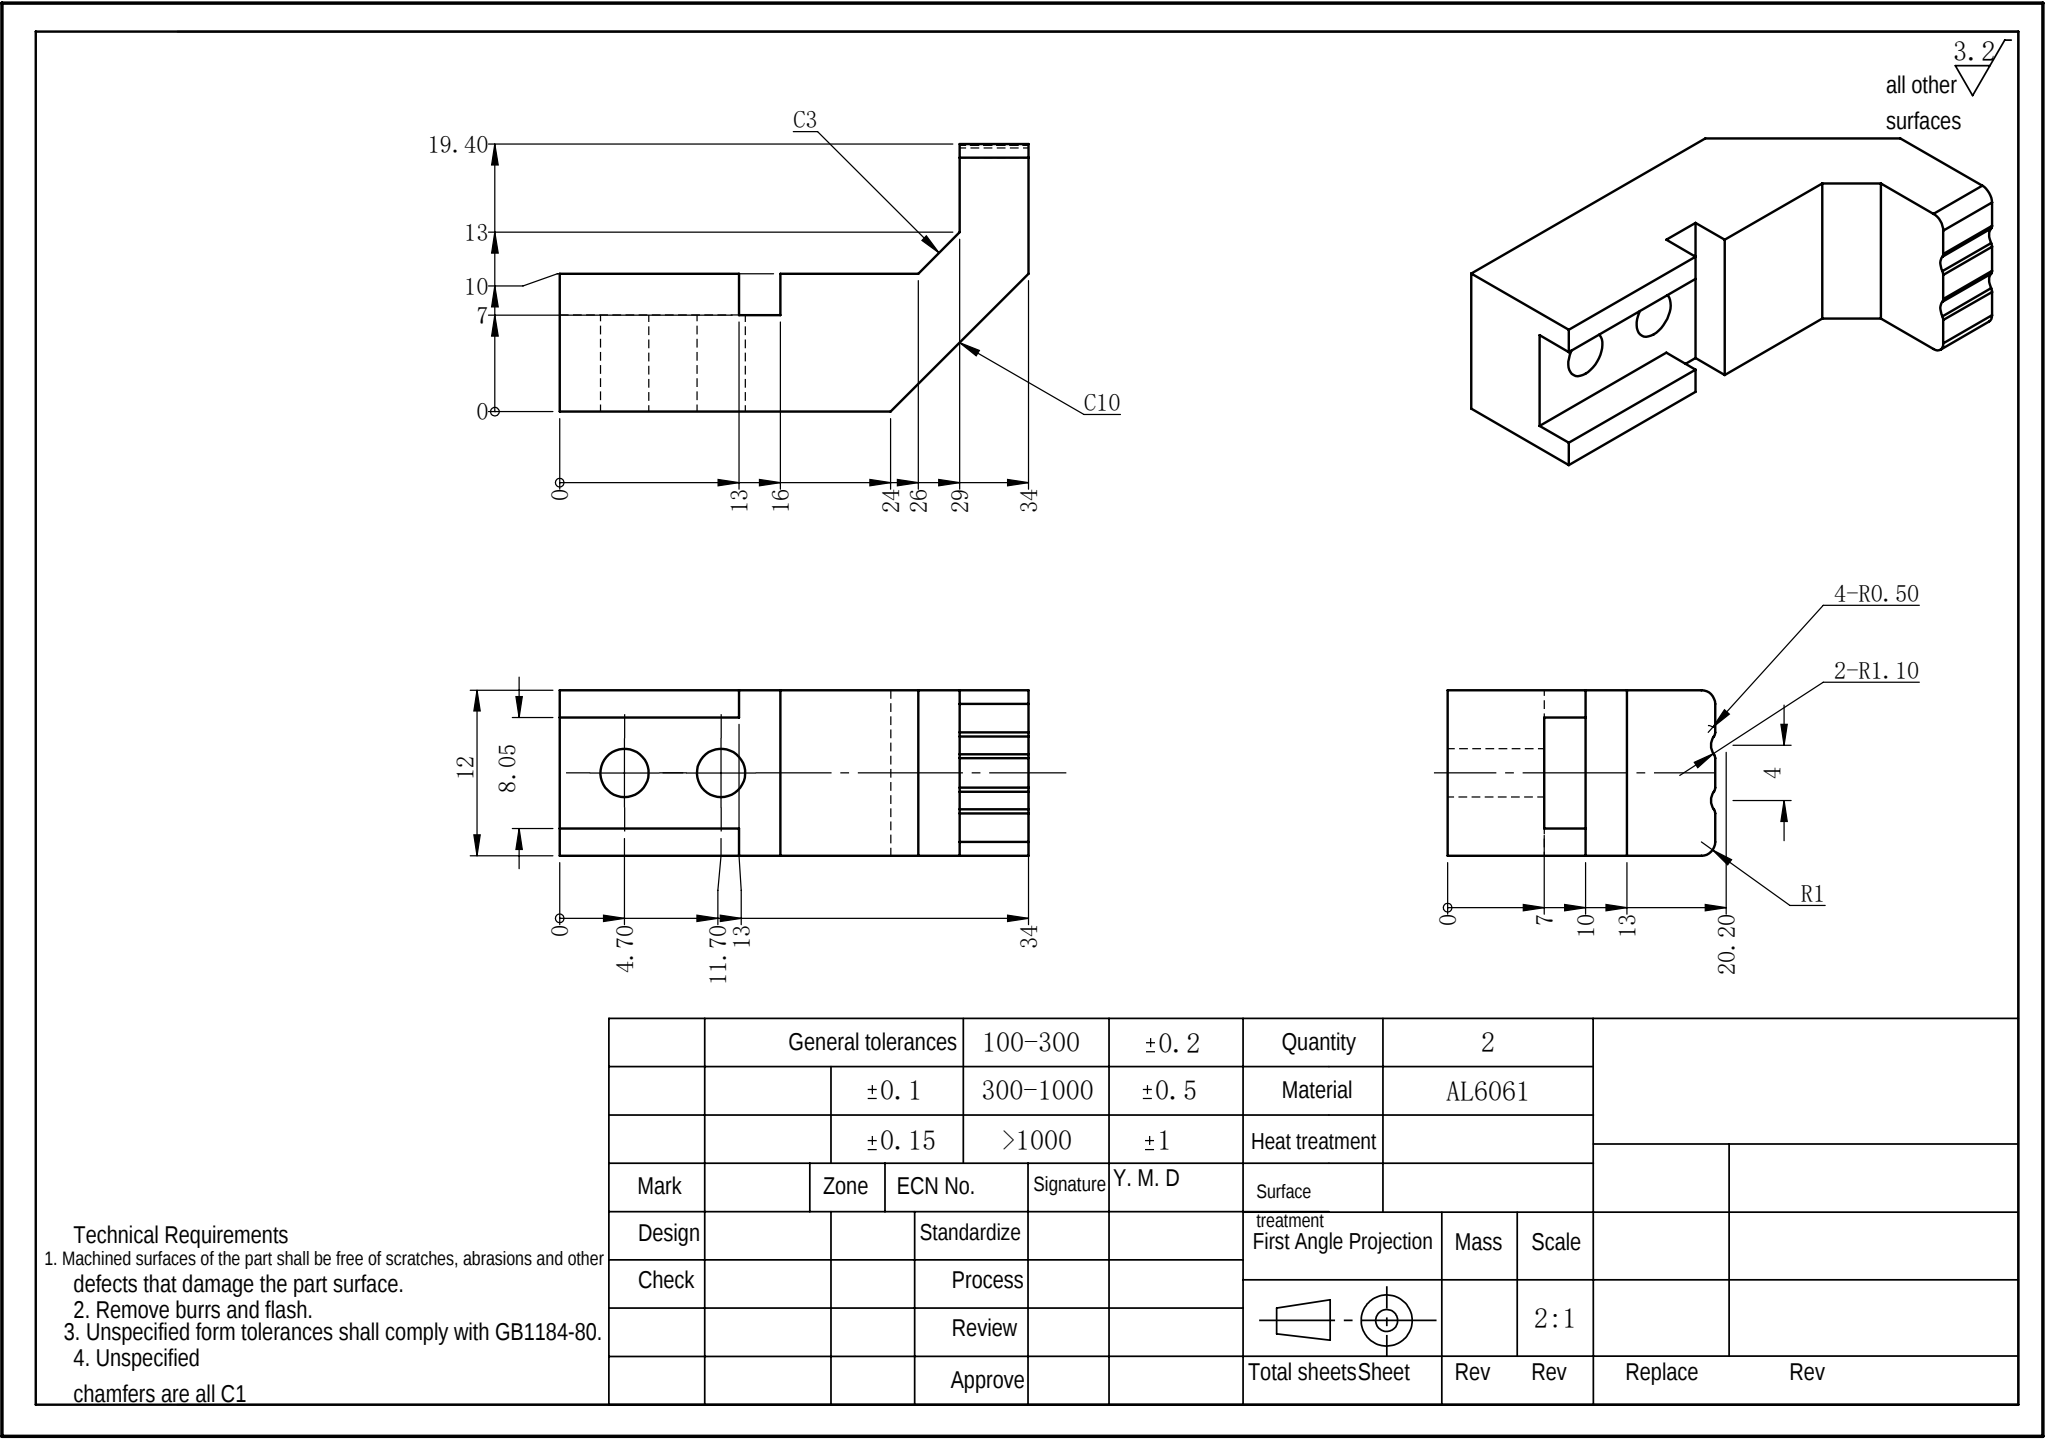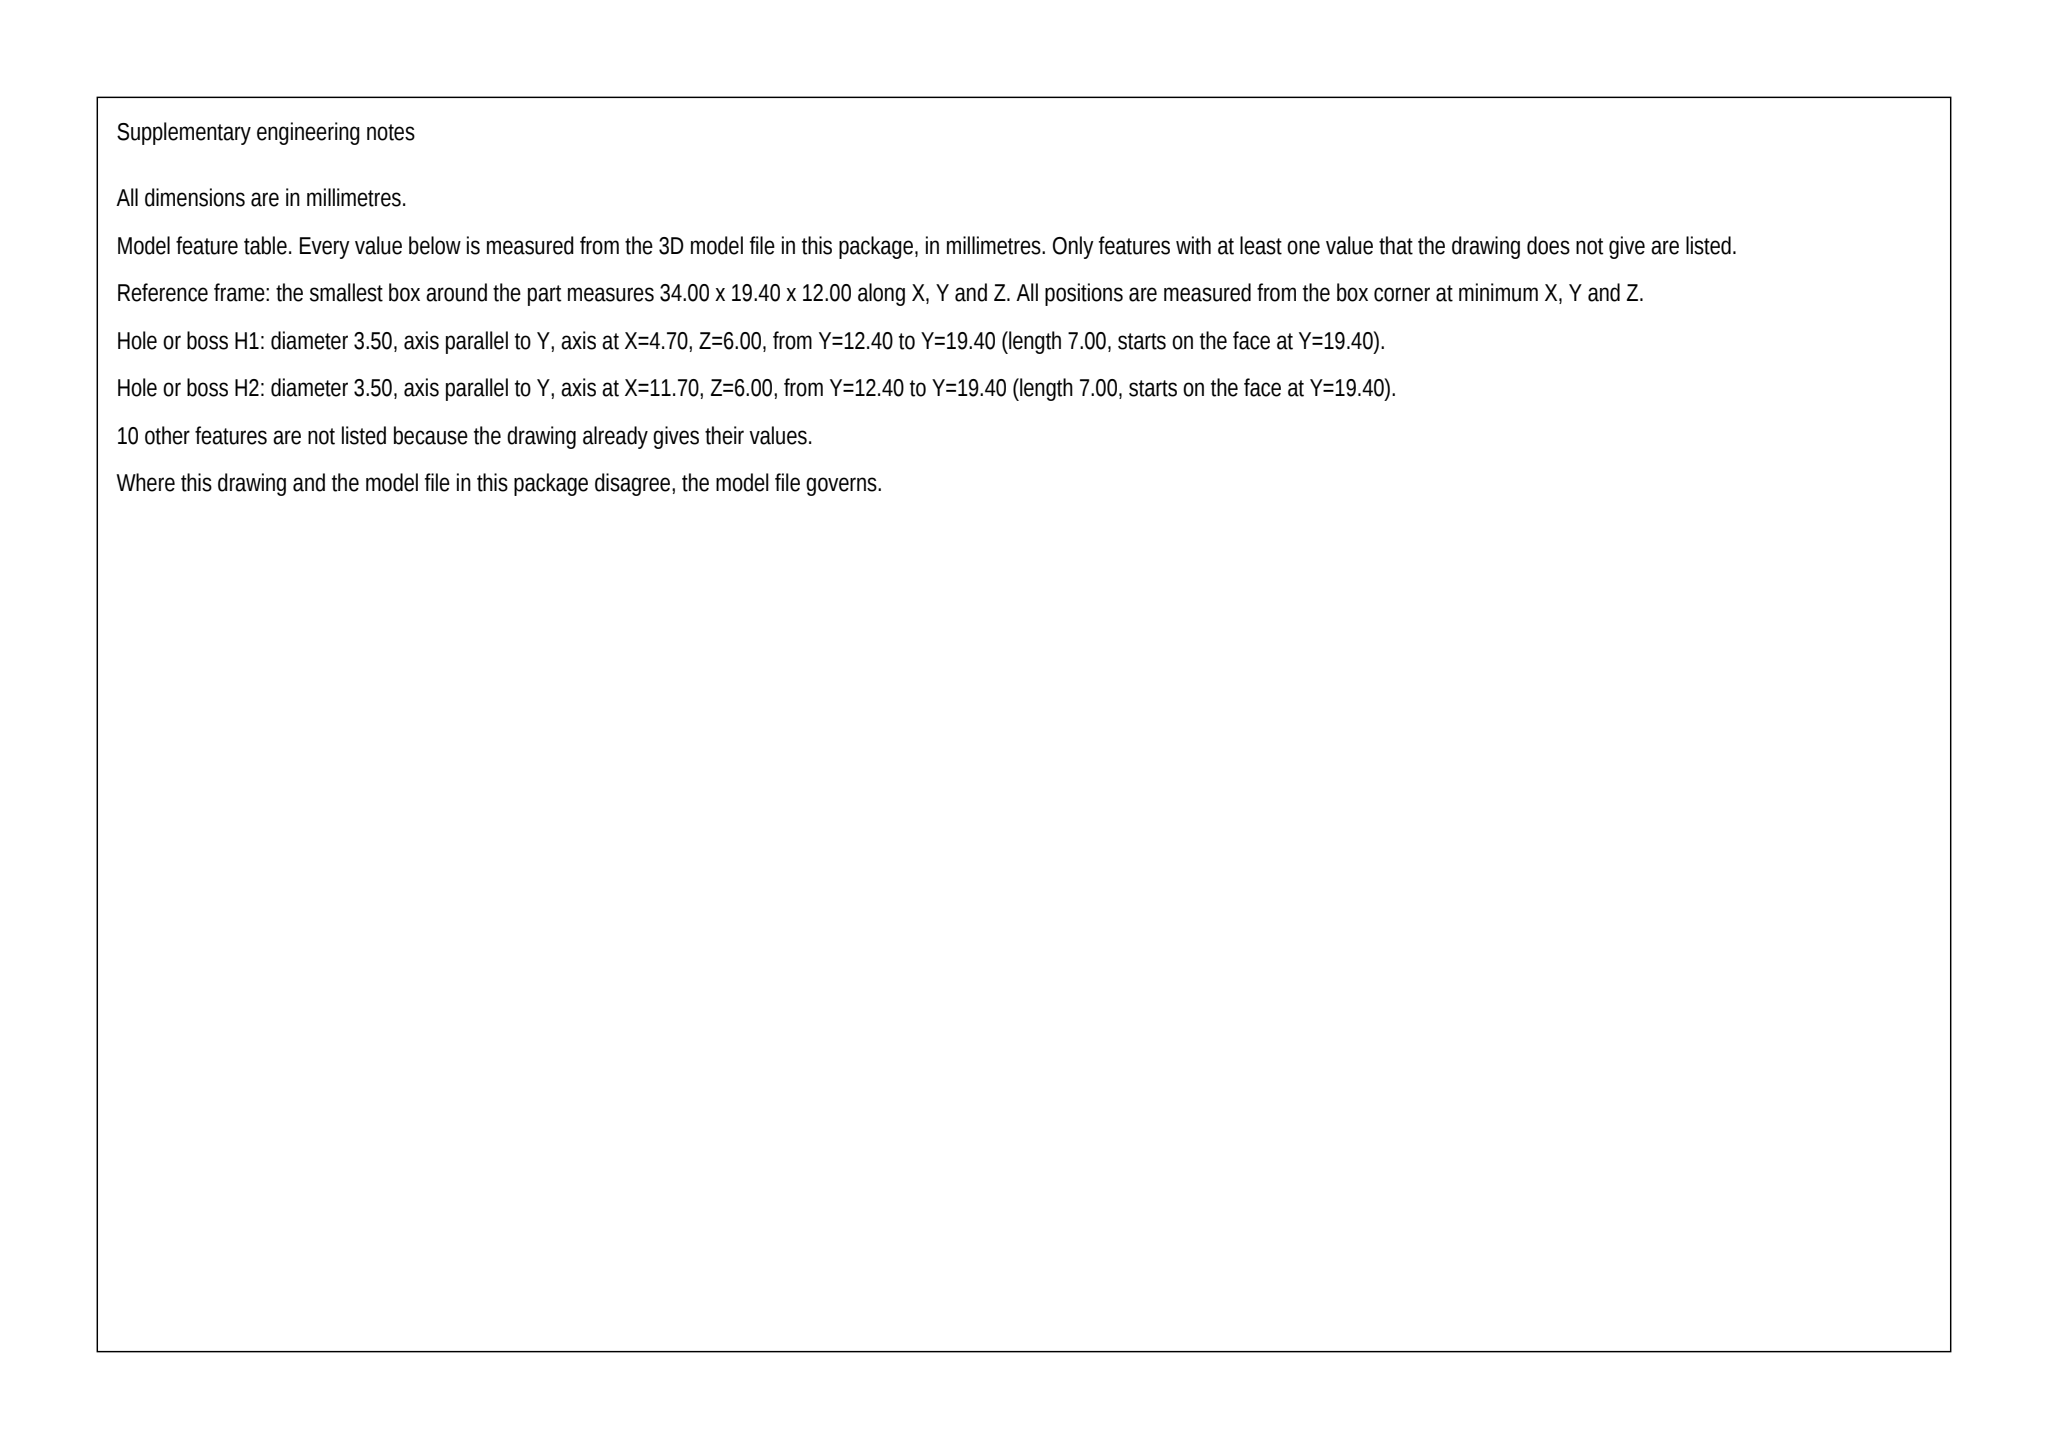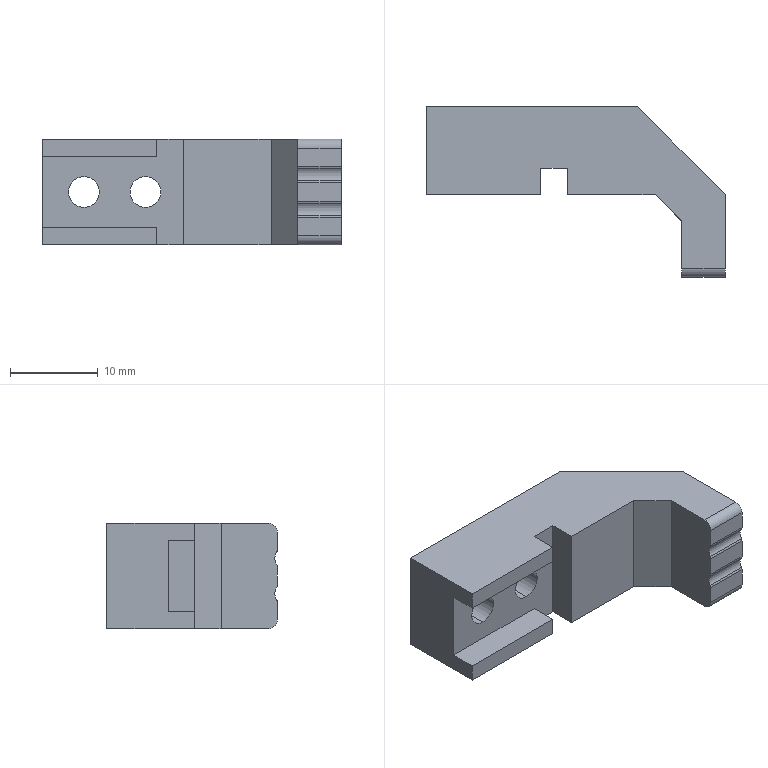Part | SolidWorks | mm | material AL6061 | 1 solid | 32 faces | box 34 x 19.4 x 12 mm | volume 3536 mm3 | plane 20 | cylinder 12 | commonest cylinder face diameters 3.5 x4 1 x4 2.2 x2 2 x2
Drawing notes:
4-R0.50 GROOVE CLS: 1.07 & 2.93 EA SIDE OF 12 WIDTH CL | from the solid: 4x dia 1.0 cyls, axis x, z = 3.07/4.93/7.07/8.93; width 12 => CL at z=6.0 (+/-1.07, +/-2.93)
4-R0.50 GROOVE CLS 0.50 FROM GROOVED END FACE (ORD 18.90) | from the solid: dia 1.0 cyls at y=0.5 from end face; face at drawing ord 19.4 (bbox y=19.4), R1.10 at y=-0.8 = ord 20.20
2-R1.10 SCALLOPS: 0.30 DEEP, ARC CTR 0.80 BELOW END FACE | from the solid: Cyl dia2.2 (R1.10), axis x, at y=-0.80, z=4.0 & 8.0; face at y=0 -> 1.10-0.80=0.30 deep, 4 apart
build123d program:
from build123d import *

# Parameters (mm, degrees)
SKETCH1_W           = 34
SKETCH1_H           = 12
BOSS_EXTRUDE1_DEPTH = 5
SKETCH2_W           = 32
SKETCH2_H           = 8.05
CUT_EXTRUDE1_DEPTH  = 3
SKETCH3_W           = 3
SKETCH3_H           = 12
CUT_EXTRUDE2_DEPTH  = 3
SKETCH4_R           = 1.75
CUT_EXTRUDE3_DEPTH  = 21.616
SKETCH5_W           = 5
SKETCH5_H           = 12
BOSS_EXTRUDE2_DEPTH = 9.4
CHAMFER1_SIZE       = 10
CHAMFER2_SIZE       = 3
SKETCH6_R           = 1.1
CUT_EXTRUDE4_DEPTH  = 6
FILLET1_R           = 0.5
FILLET2_R           = 1


with BuildPart() as part:
    # Sketch1 → Boss-Extrude1 (new, symmetric)
    with BuildSketch(Plane(origin=(0, 0, 0), x_dir=(1, 0, 0), z_dir=(0, 1, 0))):
        Rectangle(SKETCH1_W, SKETCH1_H)
    extrude(amount=BOSS_EXTRUDE1_DEPTH, both=True)

    # Sketch2 → Cut-Extrude1 (cut)
    with BuildSketch(Plane.XZ.offset(5)):
        with Locations((-17, 0)):
            Rectangle(SKETCH2_W, SKETCH2_H)
    extrude(amount=-CUT_EXTRUDE1_DEPTH, mode=Mode.SUBTRACT)

    # Sketch3 → Cut-Extrude2 (cut)
    with BuildSketch(Plane.XZ.offset(5)):
        with Locations((-2.5, 0)):
            Rectangle(SKETCH3_W, SKETCH3_H)
    extrude(amount=-CUT_EXTRUDE2_DEPTH, mode=Mode.SUBTRACT)

    # Sketch4 → Cut-Extrude3 (cut, through all)
    with BuildSketch(Plane(origin=(0, 5, 0), x_dir=(1, 0, 0), z_dir=(0, 1, 0))):
        with Locations(Location((-12.3, 0, 0), (0, 0, 270))):
            Circle(SKETCH4_R)
        with Locations(Location((-5.3, 0, 0), (0, 0, 270))):
            Circle(SKETCH4_R)
    extrude(amount=-CUT_EXTRUDE3_DEPTH, mode=Mode.SUBTRACT)

    # Sketch5 → Boss-Extrude2 (add)
    with BuildSketch(Plane.XZ.offset(5)):
        with Locations((14.5, 0)):
            Rectangle(SKETCH5_W, SKETCH5_H)
    extrude(amount=BOSS_EXTRUDE2_DEPTH)

    # Chamfer1
    chamfer1_edges = [part.edges().sort_by_distance(p)[0] for p in [
        (17, 5, 0),
    ]]
    chamfer(chamfer1_edges, length=CHAMFER1_SIZE)

    # Chamfer2
    chamfer2_edges = [part.edges().sort_by_distance(p)[0] for p in [
        (12, -5, 0),
    ]]
    chamfer(chamfer2_edges, length=CHAMFER2_SIZE)

    # Sketch6 → Cut-Extrude4 (cut)
    with BuildSketch(Plane.ZY.offset(-12)):
        with Locations((2, -15.2)):
            Circle(SKETCH6_R)
        with Locations((-2, -15.2)):
            Circle(SKETCH6_R)
    extrude(amount=-CUT_EXTRUDE4_DEPTH, mode=Mode.SUBTRACT)

    # Fillet1
    fillet1_edges = [part.edges().sort_by_distance(p)[0] for p in [
        (14.5, -14.4, 1.245),
        (14.5, -14.4, 2.755),
        (14.5, -14.4, -2.755),
        (14.5, -14.4, -1.245),
    ]]
    fillet(fillet1_edges, radius=FILLET1_R)

    # Fillet2
    fillet2_edges = [part.edges().sort_by_distance(p)[0] for p in [
        (14.5, -14.4, 6),
        (14.5, -14.4, -6),
    ]]
    fillet(fillet2_edges, radius=FILLET2_R)


solid = part.part